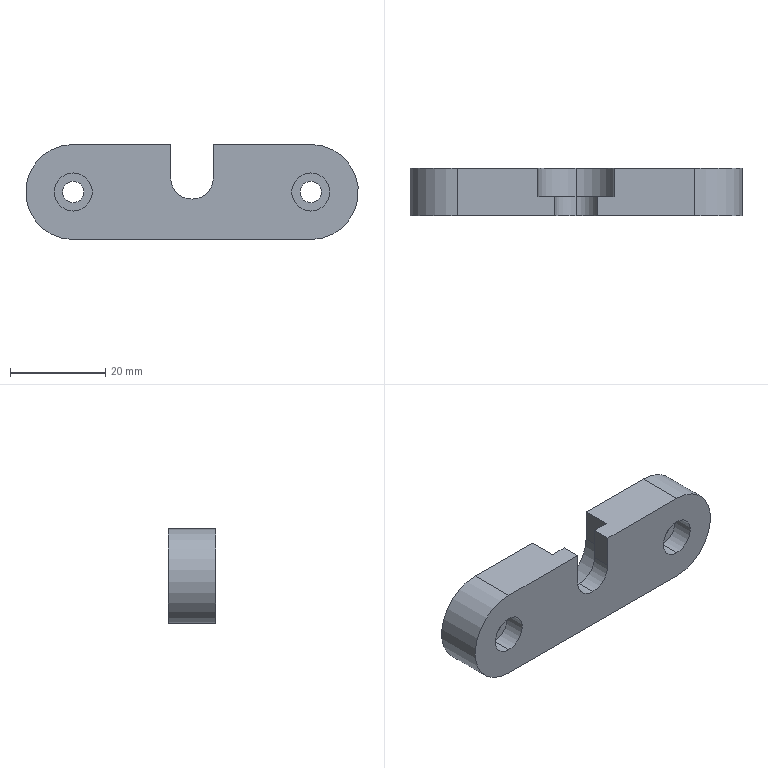Component | SolidWorks | 002MaterialPickingModuleA-1_004SidePlugModule-1_J-018-1 | 1 solid | 26 faces | box 70 x 10 x 20 mm | volume 10867 mm3 | cylinder 14 | plane 12 | commonest cylinder face diameters 8 x4 4.5 x4 9 x2 16 x2 20 x2 | material 45
build123d program:
from build123d import *

# Parameters (mm, degrees)
BOSS_EXTRUDE1_DEPTH                             = 5
M4_HEX_SOCKET_HEAD_CAP_SCREW_CBORE1_D           = 4.5
M4_HEX_SOCKET_HEAD_CAP_SCREW_CBORE1_CBORE_D     = 8
M4_HEX_SOCKET_HEAD_CAP_SCREW_CBORE1_CBORE_DEPTH = 4.4
CUT_EXTRUDE1_DEPTH                              = 6
CUT_EXTRUDE2_DEPTH                              = 37.892


with BuildPart() as part:
    # Sketch1 → Boss-Extrude1 (new, symmetric)
    with BuildSketch(Plane(origin=(0, 0, 0), x_dir=(1, 0, 0), z_dir=(0, 1, 0))):
        with BuildLine():
            Line((25, -10), (-25, -10))
            ThreePointArc((-25, -10), (-35, 0), (-25, 10))
            Line((-25, 10), (25, 10))
            ThreePointArc((25, 10), (35, 0), (25, -10))
        make_face()
    extrude(amount=BOSS_EXTRUDE1_DEPTH, both=True)

    # M4 Hex Socket Head Cap Screw CBORE1 (through all)
    with Locations(Plane(origin=(0, 5, 0), x_dir=(1, 0, 0), z_dir=(0, 1, 0))):
        with Locations((-25, 0), (25, 0)):
            CounterBoreHole(M4_HEX_SOCKET_HEAD_CAP_SCREW_CBORE1_D / 2, M4_HEX_SOCKET_HEAD_CAP_SCREW_CBORE1_CBORE_D / 2, M4_HEX_SOCKET_HEAD_CAP_SCREW_CBORE1_CBORE_DEPTH)

    # Sketch4 → Cut-Extrude1 (cut)
    with BuildSketch(Plane.XZ.offset(5)):
        with BuildLine():
            Line((8, 10), (8, 3))
            ThreePointArc((8, 3), (0, -5), (-8, 3))
            Line((-8, 3), (-8, 10))
            ThreePointArc((-8, 10), (0, 18), (8, 10))
        make_face()
    extrude(amount=-CUT_EXTRUDE1_DEPTH, mode=Mode.SUBTRACT)

    # Sketch5 → Cut-Extrude2 (cut, through all)
    with BuildSketch(Plane.XZ.offset(-1)):
        with BuildLine():
            Line((-4.5, 3), (-4.5, 10))
            ThreePointArc((-4.5, 10), (0, 14.5), (4.5, 10))
            Line((4.5, 10), (4.5, 3))
            ThreePointArc((4.5, 3), (0, -1.5), (-4.5, 3))
        make_face()
    extrude(amount=-CUT_EXTRUDE2_DEPTH, mode=Mode.SUBTRACT)


solid = part.part

# Placed as in the assembly
solid = solid.moved(Location((220.325, 273.019, 464.731), (0, 0, 180)))
STEP:
#1=COLOUR_RGB('',0.7922,0.8196,0.9333);
#2=FILL_AREA_STYLE_COLOUR('',#1);
#3=FILL_AREA_STYLE('',(#2));
#4=SURFACE_STYLE_FILL_AREA(#3);
#5=SURFACE_SIDE_STYLE('',(#4));
#6=SURFACE_STYLE_USAGE(.BOTH.,#5);
#7=PRESENTATION_STYLE_ASSIGNMENT((#6));
#8=CARTESIAN_POINT('',(8.674,10.552,18.237));
#9=VERTEX_POINT('',#8);
#10=CARTESIAN_POINT('',(8.497,10.552,18.415));
#11=VERTEX_POINT('',#10);
#12=CARTESIAN_POINT('',(8.674,10.552,18.415));
#13=DIRECTION('',(0.,1.,0.));
#14=DIRECTION('',(0.,0.,-1.));
#15=AXIS2_PLACEMENT_3D('',#12,#13,#14);
#16=CIRCLE('',#15,0.1772);
#17=EDGE_CURVE('',#9,#11,#16,.T.);
#18=ORIENTED_EDGE('',*,*,#17,.F.);
#19=CARTESIAN_POINT('',(8.674,10.709,18.237));
#20=VERTEX_POINT('',#19);
#21=CARTESIAN_POINT('',(8.674,10.552,18.237));
#22=DIRECTION('',(0.,1.,0.));
#23=VECTOR('',#22,39.37);
#24=LINE('',#21,#23);
#25=EDGE_CURVE('',#9,#20,#24,.T.);
#26=ORIENTED_EDGE('',*,*,#25,.T.);
#27=CARTESIAN_POINT('',(8.497,10.709,18.415));
#28=VERTEX_POINT('',#27);
#29=CARTESIAN_POINT('',(8.674,10.709,18.415));
#30=DIRECTION('',(0.,1.,0.));
#31=DIRECTION('',(0.,0.,-1.));
#32=AXIS2_PLACEMENT_3D('',#29,#30,#31);
#33=CIRCLE('',#32,0.1772);
#34=EDGE_CURVE('',#20,#28,#33,.T.);
#35=ORIENTED_EDGE('',*,*,#34,.T.);
#36=CARTESIAN_POINT('',(8.497,10.552,18.415));
#37=DIRECTION('',(0.,1.,0.));
#38=VECTOR('',#37,39.37);
#39=LINE('',#36,#38);
#40=EDGE_CURVE('',#11,#28,#39,.T.);
#41=ORIENTED_EDGE('',*,*,#40,.F.);
#42=EDGE_LOOP('',(#18,#26,#35,#41));
#43=FACE_OUTER_BOUND('',#42,.T.);
#44=CARTESIAN_POINT('',(8.674,10.552,18.415));
#45=DIRECTION('',(0.,1.,0.));
#46=DIRECTION('',(0.,0.,-1.));
#47=AXIS2_PLACEMENT_3D('',#44,#45,#46);
#48=CYLINDRICAL_SURFACE('',#47,0.1772);
#49=ADVANCED_FACE('',(#43),#48,.F.);
#50=CARTESIAN_POINT('',(8.674,10.709,18.1));
#51=VERTEX_POINT('',#50);
#52=CARTESIAN_POINT('',(8.359,10.709,18.415));
#53=VERTEX_POINT('',#52);
#54=CARTESIAN_POINT('',(8.674,10.709,18.415));
#55=DIRECTION('',(0.,1.,0.));
#56=DIRECTION('',(0.,0.,1.));
#57=AXIS2_PLACEMENT_3D('',#54,#55,#56);
#58=CIRCLE('',#57,0.315);
#59=EDGE_CURVE('',#51,#53,#58,.T.);
#60=ORIENTED_EDGE('',*,*,#59,.F.);
#61=CARTESIAN_POINT('',(8.674,10.946,18.1));
#62=VERTEX_POINT('',#61);
#63=CARTESIAN_POINT('',(8.674,9.449,18.1));
#64=DIRECTION('',(0.,1.,0.));
#65=VECTOR('',#64,39.37);
#66=LINE('',#63,#65);
#67=EDGE_CURVE('',#51,#62,#66,.T.);
#68=ORIENTED_EDGE('',*,*,#67,.T.);
#69=CARTESIAN_POINT('',(8.359,10.946,18.415));
#70=VERTEX_POINT('',#69);
#71=CARTESIAN_POINT('',(8.674,10.946,18.415));
#72=DIRECTION('',(0.,1.,0.));
#73=DIRECTION('',(0.,0.,-1.));
#74=AXIS2_PLACEMENT_3D('',#71,#72,#73);
#75=CIRCLE('',#74,0.315);
#76=EDGE_CURVE('',#62,#70,#75,.T.);
#77=ORIENTED_EDGE('',*,*,#76,.T.);
#78=CARTESIAN_POINT('',(8.359,9.449,18.415));
#79=DIRECTION('',(0.,1.,0.));
#80=VECTOR('',#79,39.37);
#81=LINE('',#78,#80);
#82=EDGE_CURVE('',#53,#70,#81,.T.);
#83=ORIENTED_EDGE('',*,*,#82,.F.);
#84=EDGE_LOOP('',(#60,#68,#77,#83));
#85=FACE_OUTER_BOUND('',#84,.T.);
#86=CARTESIAN_POINT('',(8.674,9.449,18.415));
#87=DIRECTION('',(0.,1.,0.));
#88=DIRECTION('',(0.,0.,-1.));
#89=AXIS2_PLACEMENT_3D('',#86,#87,#88);
#90=CYLINDRICAL_SURFACE('',#89,0.315);
#91=ADVANCED_FACE('',(#85),#90,.F.);
#92=CARTESIAN_POINT('',(9.658,10.725,18.139));
#93=VERTEX_POINT('',#92);
#94=CARTESIAN_POINT('',(9.658,10.725,18.454));
#95=VERTEX_POINT('',#94);
#96=CARTESIAN_POINT('',(9.658,10.725,18.296));
#97=DIRECTION('',(-0.,-1.,-0.));
#98=DIRECTION('',(0.,0.,1.));
#99=AXIS2_PLACEMENT_3D('',#96,#97,#98);
#100=CIRCLE('',#99,0.1575);
#101=EDGE_CURVE('',#93,#95,#100,.T.);
#102=ORIENTED_EDGE('',*,*,#101,.F.);
#103=CARTESIAN_POINT('',(9.658,10.552,18.139));
#104=VERTEX_POINT('',#103);
#105=CARTESIAN_POINT('',(9.658,10.552,18.139));
#106=DIRECTION('',(-0.,-1.,-0.));
#107=VECTOR('',#106,39.37);
#108=LINE('',#105,#107);
#109=EDGE_CURVE('',#93,#104,#108,.T.);
#110=ORIENTED_EDGE('',*,*,#109,.T.);
#111=CARTESIAN_POINT('',(9.658,10.552,18.454));
#112=VERTEX_POINT('',#111);
#113=CARTESIAN_POINT('',(9.658,10.552,18.296));
#114=DIRECTION('',(-0.,-1.,-0.));
#115=DIRECTION('',(0.,0.,1.));
#116=AXIS2_PLACEMENT_3D('',#113,#114,#115);
#117=CIRCLE('',#116,0.1575);
#118=EDGE_CURVE('',#104,#112,#117,.T.);
#119=ORIENTED_EDGE('',*,*,#118,.T.);
#120=CARTESIAN_POINT('',(9.658,10.552,18.454));
#121=DIRECTION('',(-0.,-1.,-0.));
#122=VECTOR('',#121,39.37);
#123=LINE('',#120,#122);
#124=EDGE_CURVE('',#95,#112,#123,.T.);
#125=ORIENTED_EDGE('',*,*,#124,.F.);
#126=EDGE_LOOP('',(#102,#110,#119,#125));
#127=FACE_OUTER_BOUND('',#126,.T.);
#128=CARTESIAN_POINT('',(9.658,10.552,18.296));
#129=DIRECTION('',(-0.,-1.,-0.));
#130=DIRECTION('',(0.,0.,1.));
#131=AXIS2_PLACEMENT_3D('',#128,#129,#130);
#132=CYLINDRICAL_SURFACE('',#131,0.1575);
#133=ADVANCED_FACE('',(#127),#132,.F.);
#134=CARTESIAN_POINT('',(9.658,10.946,18.208));
#135=VERTEX_POINT('',#134);
#136=CARTESIAN_POINT('',(9.658,10.946,18.385));
#137=VERTEX_POINT('',#136);
#138=CARTESIAN_POINT('',(9.658,10.946,18.296));
#139=DIRECTION('',(-0.,-1.,-0.));
#140=DIRECTION('',(0.,0.,1.));
#141=AXIS2_PLACEMENT_3D('',#138,#139,#140);
#142=CIRCLE('',#141,0.08858);
#143=EDGE_CURVE('',#135,#137,#142,.T.);
#144=ORIENTED_EDGE('',*,*,#143,.F.);
#145=CARTESIAN_POINT('',(9.658,10.725,18.208));
#146=VERTEX_POINT('',#145);
#147=CARTESIAN_POINT('',(9.658,10.552,18.208));
#148=DIRECTION('',(-0.,-1.,-0.));
#149=VECTOR('',#148,39.37);
#150=LINE('',#147,#149);
#151=EDGE_CURVE('',#135,#146,#150,.T.);
#152=ORIENTED_EDGE('',*,*,#151,.T.);
#153=CARTESIAN_POINT('',(9.658,10.725,18.385));
#154=VERTEX_POINT('',#153);
#155=CARTESIAN_POINT('',(9.658,10.725,18.296));
#156=DIRECTION('',(-0.,-1.,-0.));
#157=DIRECTION('',(0.,0.,1.));
#158=AXIS2_PLACEMENT_3D('',#155,#156,#157);
#159=CIRCLE('',#158,0.08858);
#160=EDGE_CURVE('',#146,#154,#159,.T.);
#161=ORIENTED_EDGE('',*,*,#160,.T.);
#162=CARTESIAN_POINT('',(9.658,10.552,18.385));
#163=DIRECTION('',(-0.,-1.,-0.));
#164=VECTOR('',#163,39.37);
#165=LINE('',#162,#164);
#166=EDGE_CURVE('',#137,#154,#165,.T.);
#167=ORIENTED_EDGE('',*,*,#166,.F.);
#168=EDGE_LOOP('',(#144,#152,#161,#167));
#169=FACE_OUTER_BOUND('',#168,.T.);
#170=CARTESIAN_POINT('',(9.658,10.552,18.296));
#171=DIRECTION('',(-0.,-1.,-0.));
#172=DIRECTION('',(0.,0.,1.));
#173=AXIS2_PLACEMENT_3D('',#170,#171,#172);
#174=CYLINDRICAL_SURFACE('',#173,0.08858);
#175=ADVANCED_FACE('',(#169),#174,.F.);
#176=CARTESIAN_POINT('',(7.69,10.725,18.139));
#177=VERTEX_POINT('',#176);
#178=CARTESIAN_POINT('',(7.69,10.725,18.454));
#179=VERTEX_POINT('',#178);
#180=CARTESIAN_POINT('',(7.69,10.725,18.296));
#181=DIRECTION('',(-0.,-1.,-0.));
#182=DIRECTION('',(0.,0.,1.));
#183=AXIS2_PLACEMENT_3D('',#180,#181,#182);
#184=CIRCLE('',#183,0.1575);
#185=EDGE_CURVE('',#177,#179,#184,.T.);
#186=ORIENTED_EDGE('',*,*,#185,.F.);
#187=CARTESIAN_POINT('',(7.69,10.552,18.139));
#188=VERTEX_POINT('',#187);
#189=CARTESIAN_POINT('',(7.69,10.552,18.139));
#190=DIRECTION('',(-0.,-1.,-0.));
#191=VECTOR('',#190,39.37);
#192=LINE('',#189,#191);
#193=EDGE_CURVE('',#177,#188,#192,.T.);
#194=ORIENTED_EDGE('',*,*,#193,.T.);
#195=CARTESIAN_POINT('',(7.69,10.552,18.454));
#196=VERTEX_POINT('',#195);
#197=CARTESIAN_POINT('',(7.69,10.552,18.296));
#198=DIRECTION('',(-0.,-1.,-0.));
#199=DIRECTION('',(0.,0.,1.));
#200=AXIS2_PLACEMENT_3D('',#197,#198,#199);
#201=CIRCLE('',#200,0.1575);
#202=EDGE_CURVE('',#188,#196,#201,.T.);
#203=ORIENTED_EDGE('',*,*,#202,.T.);
#204=CARTESIAN_POINT('',(7.69,10.552,18.454));
#205=DIRECTION('',(-0.,-1.,-0.));
#206=VECTOR('',#205,39.37);
#207=LINE('',#204,#206);
#208=EDGE_CURVE('',#179,#196,#207,.T.);
#209=ORIENTED_EDGE('',*,*,#208,.F.);
#210=EDGE_LOOP('',(#186,#194,#203,#209));
#211=FACE_OUTER_BOUND('',#210,.T.);
#212=CARTESIAN_POINT('',(7.69,10.552,18.296));
#213=DIRECTION('',(-0.,-1.,-0.));
#214=DIRECTION('',(0.,0.,1.));
#215=AXIS2_PLACEMENT_3D('',#212,#213,#214);
#216=CYLINDRICAL_SURFACE('',#215,0.1575);
#217=ADVANCED_FACE('',(#211),#216,.F.);
#218=CARTESIAN_POINT('',(7.69,10.946,18.208));
#219=VERTEX_POINT('',#218);
#220=CARTESIAN_POINT('',(7.69,10.946,18.385));
#221=VERTEX_POINT('',#220);
#222=CARTESIAN_POINT('',(7.69,10.946,18.296));
#223=DIRECTION('',(-0.,-1.,-0.));
#224=DIRECTION('',(0.,0.,1.));
#225=AXIS2_PLACEMENT_3D('',#222,#223,#224);
#226=CIRCLE('',#225,0.08858);
#227=EDGE_CURVE('',#219,#221,#226,.T.);
#228=ORIENTED_EDGE('',*,*,#227,.F.);
#229=CARTESIAN_POINT('',(7.69,10.725,18.208));
#230=VERTEX_POINT('',#229);
#231=CARTESIAN_POINT('',(7.69,10.552,18.208));
#232=DIRECTION('',(-0.,-1.,-0.));
#233=VECTOR('',#232,39.37);
#234=LINE('',#231,#233);
#235=EDGE_CURVE('',#219,#230,#234,.T.);
#236=ORIENTED_EDGE('',*,*,#235,.T.);
#237=CARTESIAN_POINT('',(7.69,10.725,18.385));
#238=VERTEX_POINT('',#237);
#239=CARTESIAN_POINT('',(7.69,10.725,18.296));
#240=DIRECTION('',(-0.,-1.,-0.));
#241=DIRECTION('',(0.,0.,1.));
#242=AXIS2_PLACEMENT_3D('',#239,#240,#241);
#243=CIRCLE('',#242,0.08858);
#244=EDGE_CURVE('',#230,#238,#243,.T.);
#245=ORIENTED_EDGE('',*,*,#244,.T.);
#246=CARTESIAN_POINT('',(7.69,10.552,18.385));
#247=DIRECTION('',(-0.,-1.,-0.));
#248=VECTOR('',#247,39.37);
#249=LINE('',#246,#248);
#250=EDGE_CURVE('',#221,#238,#249,.T.);
#251=ORIENTED_EDGE('',*,*,#250,.F.);
#252=EDGE_LOOP('',(#228,#236,#245,#251));
#253=FACE_OUTER_BOUND('',#252,.T.);
#254=CARTESIAN_POINT('',(7.69,10.552,18.296));
#255=DIRECTION('',(-0.,-1.,-0.));
#256=DIRECTION('',(0.,0.,1.));
#257=AXIS2_PLACEMENT_3D('',#254,#255,#256);
#258=CYLINDRICAL_SURFACE('',#257,0.08858);
#259=ADVANCED_FACE('',(#253),#258,.F.);
#260=CARTESIAN_POINT('',(8.989,10.709,18.69));
#261=VERTEX_POINT('',#260);
#262=CARTESIAN_POINT('',(8.851,10.709,18.69));
#263=VERTEX_POINT('',#262);
#264=CARTESIAN_POINT('',(7.69,10.709,18.69));
#265=DIRECTION('',(-1.,0.,-0.));
#266=VECTOR('',#265,39.37);
#267=LINE('',#264,#266);
#268=EDGE_CURVE('',#261,#263,#267,.T.);
#269=ORIENTED_EDGE('',*,*,#268,.T.);
#270=CARTESIAN_POINT('',(8.851,10.552,18.69));
#271=VERTEX_POINT('',#270);
#272=CARTESIAN_POINT('',(8.851,10.552,18.69));
#273=DIRECTION('',(0.,1.,0.));
#274=VECTOR('',#273,39.37);
#275=LINE('',#272,#274);
#276=EDGE_CURVE('',#271,#263,#275,.T.);
#277=ORIENTED_EDGE('',*,*,#276,.F.);
#278=CARTESIAN_POINT('',(9.658,10.552,18.69));
#279=VERTEX_POINT('',#278);
#280=CARTESIAN_POINT('',(7.69,10.552,18.69));
#281=DIRECTION('',(-1.,0.,-0.));
#282=VECTOR('',#281,39.37);
#283=LINE('',#280,#282);
#284=EDGE_CURVE('',#279,#271,#283,.T.);
#285=ORIENTED_EDGE('',*,*,#284,.F.);
#286=CARTESIAN_POINT('',(9.658,10.946,18.69));
#287=VERTEX_POINT('',#286);
#288=CARTESIAN_POINT('',(9.658,10.552,18.69));
#289=DIRECTION('',(0.,1.,0.));
#290=VECTOR('',#289,39.37);
#291=LINE('',#288,#290);
#292=EDGE_CURVE('',#279,#287,#291,.T.);
#293=ORIENTED_EDGE('',*,*,#292,.T.);
#294=CARTESIAN_POINT('',(8.989,10.946,18.69));
#295=VERTEX_POINT('',#294);
#296=CARTESIAN_POINT('',(7.69,10.946,18.69));
#297=DIRECTION('',(-1.,0.,-0.));
#298=VECTOR('',#297,39.37);
#299=LINE('',#296,#298);
#300=EDGE_CURVE('',#287,#295,#299,.T.);
#301=ORIENTED_EDGE('',*,*,#300,.T.);
#302=CARTESIAN_POINT('',(8.989,9.449,18.69));
#303=DIRECTION('',(0.,1.,0.));
#304=VECTOR('',#303,39.37);
#305=LINE('',#302,#304);
#306=EDGE_CURVE('',#261,#295,#305,.T.);
#307=ORIENTED_EDGE('',*,*,#306,.F.);
#308=EDGE_LOOP('',(#269,#277,#285,#293,#301,#307));
#309=FACE_OUTER_BOUND('',#308,.T.);
#310=CARTESIAN_POINT('',(7.69,10.552,18.69));
#311=DIRECTION('',(0.,0.,-1.));
#312=DIRECTION('',(1.,-0.,0.));
#313=AXIS2_PLACEMENT_3D('',#310,#311,#312);
#314=PLANE('',#313);
#315=ADVANCED_FACE('',(#309),#314,.F.);
#316=CARTESIAN_POINT('',(7.69,10.946,18.69));
#317=VERTEX_POINT('',#316);
#318=CARTESIAN_POINT('',(7.69,10.946,17.903));
#319=VERTEX_POINT('',#318);
#320=CARTESIAN_POINT('',(7.69,10.946,18.296));
#321=DIRECTION('',(-0.,-1.,-0.));
#322=DIRECTION('',(0.,0.,1.));
#323=AXIS2_PLACEMENT_3D('',#320,#321,#322);
#324=CIRCLE('',#323,0.3937);
#325=EDGE_CURVE('',#317,#319,#324,.T.);
#326=ORIENTED_EDGE('',*,*,#325,.T.);
#327=CARTESIAN_POINT('',(7.69,10.552,17.903));
#328=VERTEX_POINT('',#327);
#329=CARTESIAN_POINT('',(7.69,10.552,17.903));
#330=DIRECTION('',(0.,1.,0.));
#331=VECTOR('',#330,39.37);
#332=LINE('',#329,#331);
#333=EDGE_CURVE('',#328,#319,#332,.T.);
#334=ORIENTED_EDGE('',*,*,#333,.F.);
#335=CARTESIAN_POINT('',(7.69,10.552,18.69));
#336=VERTEX_POINT('',#335);
#337=CARTESIAN_POINT('',(7.69,10.552,18.296));
#338=DIRECTION('',(-0.,-1.,-0.));
#339=DIRECTION('',(0.,0.,1.));
#340=AXIS2_PLACEMENT_3D('',#337,#338,#339);
#341=CIRCLE('',#340,0.3937);
#342=EDGE_CURVE('',#336,#328,#341,.T.);
#343=ORIENTED_EDGE('',*,*,#342,.F.);
#344=CARTESIAN_POINT('',(7.69,10.552,18.69));
#345=DIRECTION('',(0.,1.,0.));
#346=VECTOR('',#345,39.37);
#347=LINE('',#344,#346);
#348=EDGE_CURVE('',#336,#317,#347,.T.);
#349=ORIENTED_EDGE('',*,*,#348,.T.);
#350=EDGE_LOOP('',(#326,#334,#343,#349));
#351=FACE_OUTER_BOUND('',#350,.T.);
#352=CARTESIAN_POINT('',(7.69,10.552,18.296));
#353=DIRECTION('',(0.,1.,0.));
#354=DIRECTION('',(0.,0.,-1.));
#355=AXIS2_PLACEMENT_3D('',#352,#353,#354);
#356=CYLINDRICAL_SURFACE('',#355,0.3937);
#357=ADVANCED_FACE('',(#351),#356,.T.);
#358=CARTESIAN_POINT('',(9.658,10.946,17.903));
#359=VERTEX_POINT('',#358);
#360=CARTESIAN_POINT('',(7.69,10.946,17.903));
#361=DIRECTION('',(1.,-0.,0.));
#362=VECTOR('',#361,39.37);
#363=LINE('',#360,#362);
#364=EDGE_CURVE('',#319,#359,#363,.T.);
#365=ORIENTED_EDGE('',*,*,#364,.T.);
#366=CARTESIAN_POINT('',(9.658,10.552,17.903));
#367=VERTEX_POINT('',#366);
#368=CARTESIAN_POINT('',(9.658,10.552,17.903));
#369=DIRECTION('',(0.,1.,0.));
#370=VECTOR('',#369,39.37);
#371=LINE('',#368,#370);
#372=EDGE_CURVE('',#367,#359,#371,.T.);
#373=ORIENTED_EDGE('',*,*,#372,.F.);
#374=CARTESIAN_POINT('',(7.69,10.552,17.903));
#375=DIRECTION('',(1.,-0.,0.));
#376=VECTOR('',#375,39.37);
#377=LINE('',#374,#376);
#378=EDGE_CURVE('',#328,#367,#377,.T.);
#379=ORIENTED_EDGE('',*,*,#378,.F.);
#380=ORIENTED_EDGE('',*,*,#333,.T.);
#381=EDGE_LOOP('',(#365,#373,#379,#380));
#382=FACE_OUTER_BOUND('',#381,.T.);
#383=CARTESIAN_POINT('',(7.69,10.552,17.903));
#384=DIRECTION('',(-0.,-0.,1.));
#385=DIRECTION('',(-1.,0.,-0.));
#386=AXIS2_PLACEMENT_3D('',#383,#384,#385);
#387=PLANE('',#386);
#388=ADVANCED_FACE('',(#382),#387,.F.);
#389=CARTESIAN_POINT('',(9.658,10.946,18.296));
#390=DIRECTION('',(-0.,-1.,-0.));
#391=DIRECTION('',(0.,0.,1.));
#392=AXIS2_PLACEMENT_3D('',#389,#390,#391);
#393=CIRCLE('',#392,0.3937);
#394=EDGE_CURVE('',#359,#287,#393,.T.);
#395=ORIENTED_EDGE('',*,*,#394,.T.);
#396=ORIENTED_EDGE('',*,*,#292,.F.);
#397=CARTESIAN_POINT('',(9.658,10.552,18.296));
#398=DIRECTION('',(-0.,-1.,-0.));
#399=DIRECTION('',(0.,0.,1.));
#400=AXIS2_PLACEMENT_3D('',#397,#398,#399);
#401=CIRCLE('',#400,0.3937);
#402=EDGE_CURVE('',#367,#279,#401,.T.);
#403=ORIENTED_EDGE('',*,*,#402,.F.);
#404=ORIENTED_EDGE('',*,*,#372,.T.);
#405=EDGE_LOOP('',(#395,#396,#403,#404));
#406=FACE_OUTER_BOUND('',#405,.T.);
#407=CARTESIAN_POINT('',(9.658,10.552,18.296));
#408=DIRECTION('',(0.,1.,0.));
#409=DIRECTION('',(0.,0.,-1.));
#410=AXIS2_PLACEMENT_3D('',#407,#408,#409);
#411=CYLINDRICAL_SURFACE('',#410,0.3937);
#412=ADVANCED_FACE('',(#406),#411,.T.);
#413=CARTESIAN_POINT('',(8.497,10.552,18.69));
#414=VERTEX_POINT('',#413);
#415=CARTESIAN_POINT('',(7.69,10.552,18.69));
#416=DIRECTION('',(-1.,0.,-0.));
#417=VECTOR('',#416,39.37);
#418=LINE('',#415,#417);
#419=EDGE_CURVE('',#414,#336,#418,.T.);
#420=ORIENTED_EDGE('',*,*,#419,.F.);
#421=CARTESIAN_POINT('',(8.497,10.709,18.69));
#422=VERTEX_POINT('',#421);
#423=CARTESIAN_POINT('',(8.497,10.552,18.69));
#424=DIRECTION('',(0.,1.,0.));
#425=VECTOR('',#424,39.37);
#426=LINE('',#423,#425);
#427=EDGE_CURVE('',#414,#422,#426,.T.);
#428=ORIENTED_EDGE('',*,*,#427,.T.);
#429=CARTESIAN_POINT('',(8.359,10.709,18.69));
#430=VERTEX_POINT('',#429);
#431=CARTESIAN_POINT('',(7.69,10.709,18.69));
#432=DIRECTION('',(-1.,0.,-0.));
#433=VECTOR('',#432,39.37);
#434=LINE('',#431,#433);
#435=EDGE_CURVE('',#422,#430,#434,.T.);
#436=ORIENTED_EDGE('',*,*,#435,.T.);
#437=CARTESIAN_POINT('',(8.359,10.946,18.69));
#438=VERTEX_POINT('',#437);
#439=CARTESIAN_POINT('',(8.359,9.449,18.69));
#440=DIRECTION('',(0.,1.,0.));
#441=VECTOR('',#440,39.37);
#442=LINE('',#439,#441);
#443=EDGE_CURVE('',#430,#438,#442,.T.);
#444=ORIENTED_EDGE('',*,*,#443,.T.);
#445=CARTESIAN_POINT('',(7.69,10.946,18.69));
#446=DIRECTION('',(-1.,0.,-0.));
#447=VECTOR('',#446,39.37);
#448=LINE('',#445,#447);
#449=EDGE_CURVE('',#438,#317,#448,.T.);
#450=ORIENTED_EDGE('',*,*,#449,.T.);
#451=ORIENTED_EDGE('',*,*,#348,.F.);
#452=EDGE_LOOP('',(#420,#428,#436,#444,#450,#451));
#453=FACE_OUTER_BOUND('',#452,.T.);
#454=CARTESIAN_POINT('',(7.69,10.552,18.69));
#455=DIRECTION('',(0.,0.,-1.));
#456=DIRECTION('',(1.,-0.,0.));
#457=AXIS2_PLACEMENT_3D('',#454,#455,#456);
#458=PLANE('',#457);
#459=ADVANCED_FACE('',(#453),#458,.F.);
#460=CARTESIAN_POINT('',(8.851,10.552,18.415));
#461=VERTEX_POINT('',#460);
#462=CARTESIAN_POINT('',(8.851,10.552,18.415));
#463=DIRECTION('',(0.,0.,-1.));
#464=VECTOR('',#463,39.37);
#465=LINE('',#462,#464);
#466=EDGE_CURVE('',#271,#461,#465,.T.);
#467=ORIENTED_EDGE('',*,*,#466,.T.);
#468=CARTESIAN_POINT('',(8.674,10.552,18.415));
#469=DIRECTION('',(0.,1.,0.));
#470=DIRECTION('',(0.,0.,-1.));
#471=AXIS2_PLACEMENT_3D('',#468,#469,#470);
#472=CIRCLE('',#471,0.1772);
#473=EDGE_CURVE('',#461,#9,#472,.T.);
#474=ORIENTED_EDGE('',*,*,#473,.T.);
#475=ORIENTED_EDGE('',*,*,#17,.T.);
#476=CARTESIAN_POINT('',(8.497,10.552,18.415));
#477=DIRECTION('',(-0.,-0.,1.));
#478=VECTOR('',#477,39.37);
#479=LINE('',#476,#478);
#480=EDGE_CURVE('',#11,#414,#479,.T.);
#481=ORIENTED_EDGE('',*,*,#480,.T.);
#482=ORIENTED_EDGE('',*,*,#419,.T.);
#483=ORIENTED_EDGE('',*,*,#342,.T.);
#484=ORIENTED_EDGE('',*,*,#378,.T.);
#485=ORIENTED_EDGE('',*,*,#402,.T.);
#486=ORIENTED_EDGE('',*,*,#284,.T.);
#487=EDGE_LOOP('',(#467,#474,#475,#481,#482,#483,#484,#485,#486));
#488=FACE_OUTER_BOUND('',#487,.T.);
#489=CARTESIAN_POINT('',(9.658,10.552,18.296));
#490=DIRECTION('',(-0.,-1.,-0.));
#491=DIRECTION('',(0.,0.,1.));
#492=AXIS2_PLACEMENT_3D('',#489,#490,#491);
#493=CIRCLE('',#492,0.1575);
#494=EDGE_CURVE('',#112,#104,#493,.T.);
#495=ORIENTED_EDGE('',*,*,#494,.F.);
#496=ORIENTED_EDGE('',*,*,#118,.F.);
#497=EDGE_LOOP('',(#495,#496));
#498=FACE_BOUND('',#497,.T.);
#499=CARTESIAN_POINT('',(7.69,10.552,18.296));
#500=DIRECTION('',(-0.,-1.,-0.));
#501=DIRECTION('',(0.,0.,1.));
#502=AXIS2_PLACEMENT_3D('',#499,#500,#501);
#503=CIRCLE('',#502,0.1575);
#504=EDGE_CURVE('',#196,#188,#503,.T.);
#505=ORIENTED_EDGE('',*,*,#504,.F.);
#506=ORIENTED_EDGE('',*,*,#202,.F.);
#507=EDGE_LOOP('',(#505,#506));
#508=FACE_BOUND('',#507,.T.);
#509=CARTESIAN_POINT('',(7.69,10.552,18.296));
#510=DIRECTION('',(-0.,-1.,-0.));
#511=DIRECTION('',(-0.,-0.,1.));
#512=AXIS2_PLACEMENT_3D('',#509,#510,#511);
#513=PLANE('',#512);
#514=ADVANCED_FACE('',(#488,#498,#508),#513,.T.);
#515=CARTESIAN_POINT('',(9.658,10.946,18.296));
#516=DIRECTION('',(-0.,-1.,-0.));
#517=DIRECTION('',(0.,0.,1.));
#518=AXIS2_PLACEMENT_3D('',#515,#516,#517);
#519=CIRCLE('',#518,0.08858);
#520=EDGE_CURVE('',#137,#135,#519,.T.);
#521=ORIENTED_EDGE('',*,*,#520,.T.);
#522=ORIENTED_EDGE('',*,*,#143,.T.);
#523=EDGE_LOOP('',(#521,#522));
#524=FACE_BOUND('',#523,.T.);
#525=CARTESIAN_POINT('',(7.69,10.946,18.296));
#526=DIRECTION('',(-0.,-1.,-0.));
#527=DIRECTION('',(0.,0.,1.));
#528=AXIS2_PLACEMENT_3D('',#525,#526,#527);
#529=CIRCLE('',#528,0.08858);
#530=EDGE_CURVE('',#221,#219,#529,.T.);
#531=ORIENTED_EDGE('',*,*,#530,.T.);
#532=ORIENTED_EDGE('',*,*,#227,.T.);
#533=EDGE_LOOP('',(#531,#532));
#534=FACE_BOUND('',#533,.T.);
#535=CARTESIAN_POINT('',(8.989,10.946,18.415));
#536=VERTEX_POINT('',#535);
#537=CARTESIAN_POINT('',(8.674,10.946,18.415));
#538=DIRECTION('',(0.,1.,0.));
#539=DIRECTION('',(0.,0.,-1.));
#540=AXIS2_PLACEMENT_3D('',#537,#538,#539);
#541=CIRCLE('',#540,0.315);
#542=EDGE_CURVE('',#536,#62,#541,.T.);
#543=ORIENTED_EDGE('',*,*,#542,.F.);
#544=CARTESIAN_POINT('',(8.989,10.946,18.69));
#545=DIRECTION('',(-0.,0.,-1.));
#546=VECTOR('',#545,39.37);
#547=LINE('',#544,#546);
#548=EDGE_CURVE('',#295,#536,#547,.T.);
#549=ORIENTED_EDGE('',*,*,#548,.F.);
#550=ORIENTED_EDGE('',*,*,#300,.F.);
#551=ORIENTED_EDGE('',*,*,#394,.F.);
#552=ORIENTED_EDGE('',*,*,#364,.F.);
#553=ORIENTED_EDGE('',*,*,#325,.F.);
#554=ORIENTED_EDGE('',*,*,#449,.F.);
#555=CARTESIAN_POINT('',(8.359,10.946,18.69));
#556=DIRECTION('',(0.,-0.,1.));
#557=VECTOR('',#556,39.37);
#558=LINE('',#555,#557);
#559=EDGE_CURVE('',#70,#438,#558,.T.);
#560=ORIENTED_EDGE('',*,*,#559,.F.);
#561=ORIENTED_EDGE('',*,*,#76,.F.);
#562=EDGE_LOOP('',(#543,#549,#550,#551,#552,#553,#554,#560,#561));
#563=FACE_OUTER_BOUND('',#562,.T.);
#564=CARTESIAN_POINT('',(7.69,10.946,18.296));
#565=DIRECTION('',(-0.,-1.,-0.));
#566=DIRECTION('',(-0.,-0.,1.));
#567=AXIS2_PLACEMENT_3D('',#564,#565,#566);
#568=PLANE('',#567);
#569=ADVANCED_FACE('',(#524,#534,#563),#568,.F.);
#570=ORIENTED_EDGE('',*,*,#235,.F.);
#571=ORIENTED_EDGE('',*,*,#530,.F.);
#572=ORIENTED_EDGE('',*,*,#250,.T.);
#573=CARTESIAN_POINT('',(7.69,10.725,18.296));
#574=DIRECTION('',(-0.,-1.,-0.));
#575=DIRECTION('',(0.,0.,1.));
#576=AXIS2_PLACEMENT_3D('',#573,#574,#575);
#577=CIRCLE('',#576,0.08858);
#578=EDGE_CURVE('',#238,#230,#577,.T.);
#579=ORIENTED_EDGE('',*,*,#578,.T.);
#580=EDGE_LOOP('',(#570,#571,#572,#579));
#581=FACE_OUTER_BOUND('',#580,.T.);
#582=CARTESIAN_POINT('',(7.69,10.552,18.296));
#583=DIRECTION('',(-0.,-1.,-0.));
#584=DIRECTION('',(0.,0.,1.));
#585=AXIS2_PLACEMENT_3D('',#582,#583,#584);
#586=CYLINDRICAL_SURFACE('',#585,0.08858);
#587=ADVANCED_FACE('',(#581),#586,.F.);
#588=ORIENTED_EDGE('',*,*,#578,.F.);
#589=ORIENTED_EDGE('',*,*,#244,.F.);
#590=EDGE_LOOP('',(#588,#589));
#591=FACE_BOUND('',#590,.T.);
#592=CARTESIAN_POINT('',(7.69,10.725,18.296));
#593=DIRECTION('',(-0.,-1.,-0.));
#594=DIRECTION('',(0.,0.,1.));
#595=AXIS2_PLACEMENT_3D('',#592,#593,#594);
#596=CIRCLE('',#595,0.1575);
#597=EDGE_CURVE('',#179,#177,#596,.T.);
#598=ORIENTED_EDGE('',*,*,#597,.T.);
#599=ORIENTED_EDGE('',*,*,#185,.T.);
#600=EDGE_LOOP('',(#598,#599));
#601=FACE_OUTER_BOUND('',#600,.T.);
#602=CARTESIAN_POINT('',(7.601,10.725,18.296));
#603=DIRECTION('',(0.,1.,0.));
#604=DIRECTION('',(0.,0.,-1.));
#605=AXIS2_PLACEMENT_3D('',#602,#603,#604);
#606=PLANE('',#605);
#607=ADVANCED_FACE('',(#591,#601),#606,.F.);
#608=ORIENTED_EDGE('',*,*,#193,.F.);
#609=ORIENTED_EDGE('',*,*,#597,.F.);
#610=ORIENTED_EDGE('',*,*,#208,.T.);
#611=ORIENTED_EDGE('',*,*,#504,.T.);
#612=EDGE_LOOP('',(#608,#609,#610,#611));
#613=FACE_OUTER_BOUND('',#612,.T.);
#614=CARTESIAN_POINT('',(7.69,10.552,18.296));
#615=DIRECTION('',(-0.,-1.,-0.));
#616=DIRECTION('',(0.,0.,1.));
#617=AXIS2_PLACEMENT_3D('',#614,#615,#616);
#618=CYLINDRICAL_SURFACE('',#617,0.1575);
#619=ADVANCED_FACE('',(#613),#618,.F.);
#620=ORIENTED_EDGE('',*,*,#151,.F.);
#621=ORIENTED_EDGE('',*,*,#520,.F.);
#622=ORIENTED_EDGE('',*,*,#166,.T.);
#623=CARTESIAN_POINT('',(9.658,10.725,18.296));
#624=DIRECTION('',(-0.,-1.,-0.));
#625=DIRECTION('',(0.,0.,1.));
#626=AXIS2_PLACEMENT_3D('',#623,#624,#625);
#627=CIRCLE('',#626,0.08858);
#628=EDGE_CURVE('',#154,#146,#627,.T.);
#629=ORIENTED_EDGE('',*,*,#628,.T.);
#630=EDGE_LOOP('',(#620,#621,#622,#629));
#631=FACE_OUTER_BOUND('',#630,.T.);
#632=CARTESIAN_POINT('',(9.658,10.552,18.296));
#633=DIRECTION('',(-0.,-1.,-0.));
#634=DIRECTION('',(0.,0.,1.));
#635=AXIS2_PLACEMENT_3D('',#632,#633,#634);
#636=CYLINDRICAL_SURFACE('',#635,0.08858);
#637=ADVANCED_FACE('',(#631),#636,.F.);
#638=ORIENTED_EDGE('',*,*,#628,.F.);
#639=ORIENTED_EDGE('',*,*,#160,.F.);
#640=EDGE_LOOP('',(#638,#639));
#641=FACE_BOUND('',#640,.T.);
#642=CARTESIAN_POINT('',(9.658,10.725,18.296));
#643=DIRECTION('',(-0.,-1.,-0.));
#644=DIRECTION('',(0.,0.,1.));
#645=AXIS2_PLACEMENT_3D('',#642,#643,#644);
#646=CIRCLE('',#645,0.1575);
#647=EDGE_CURVE('',#95,#93,#646,.T.);
#648=ORIENTED_EDGE('',*,*,#647,.T.);
#649=ORIENTED_EDGE('',*,*,#101,.T.);
#650=EDGE_LOOP('',(#648,#649));
#651=FACE_OUTER_BOUND('',#650,.T.);
#652=CARTESIAN_POINT('',(9.57,10.725,18.296));
#653=DIRECTION('',(0.,1.,0.));
#654=DIRECTION('',(0.,0.,-1.));
#655=AXIS2_PLACEMENT_3D('',#652,#653,#654);
#656=PLANE('',#655);
#657=ADVANCED_FACE('',(#641,#651),#656,.F.);
#658=ORIENTED_EDGE('',*,*,#109,.F.);
#659=ORIENTED_EDGE('',*,*,#647,.F.);
#660=ORIENTED_EDGE('',*,*,#124,.T.);
#661=ORIENTED_EDGE('',*,*,#494,.T.);
#662=EDGE_LOOP('',(#658,#659,#660,#661));
#663=FACE_OUTER_BOUND('',#662,.T.);
#664=CARTESIAN_POINT('',(9.658,10.552,18.296));
#665=DIRECTION('',(-0.,-1.,-0.));
#666=DIRECTION('',(0.,0.,1.));
#667=AXIS2_PLACEMENT_3D('',#664,#665,#666);
#668=CYLINDRICAL_SURFACE('',#667,0.1575);
#669=ADVANCED_FACE('',(#663),#668,.F.);
#670=CARTESIAN_POINT('',(8.851,10.709,18.415));
#671=VERTEX_POINT('',#670);
#672=CARTESIAN_POINT('',(8.674,10.709,18.415));
#673=DIRECTION('',(0.,1.,0.));
#674=DIRECTION('',(0.,0.,-1.));
#675=AXIS2_PLACEMENT_3D('',#672,#673,#674);
#676=CIRCLE('',#675,0.1772);
#677=EDGE_CURVE('',#671,#20,#676,.T.);
#678=ORIENTED_EDGE('',*,*,#677,.F.);
#679=CARTESIAN_POINT('',(8.851,10.709,18.415));
#680=DIRECTION('',(0.,0.,-1.));
#681=VECTOR('',#680,39.37);
#682=LINE('',#679,#681);
#683=EDGE_CURVE('',#263,#671,#682,.T.);
#684=ORIENTED_EDGE('',*,*,#683,.F.);
#685=ORIENTED_EDGE('',*,*,#268,.F.);
#686=CARTESIAN_POINT('',(8.989,10.709,18.415));
#687=VERTEX_POINT('',#686);
#688=CARTESIAN_POINT('',(8.989,10.709,18.69));
#689=DIRECTION('',(-0.,0.,-1.));
#690=VECTOR('',#689,39.37);
#691=LINE('',#688,#690);
#692=EDGE_CURVE('',#261,#687,#691,.T.);
#693=ORIENTED_EDGE('',*,*,#692,.T.);
#694=CARTESIAN_POINT('',(8.674,10.709,18.415));
#695=DIRECTION('',(0.,1.,0.));
#696=DIRECTION('',(0.,0.,1.));
#697=AXIS2_PLACEMENT_3D('',#694,#695,#696);
#698=CIRCLE('',#697,0.315);
#699=EDGE_CURVE('',#687,#51,#698,.T.);
#700=ORIENTED_EDGE('',*,*,#699,.T.);
#701=ORIENTED_EDGE('',*,*,#59,.T.);
#702=CARTESIAN_POINT('',(8.359,10.709,18.69));
#703=DIRECTION('',(0.,-0.,1.));
#704=VECTOR('',#703,39.37);
#705=LINE('',#702,#704);
#706=EDGE_CURVE('',#53,#430,#705,.T.);
#707=ORIENTED_EDGE('',*,*,#706,.T.);
#708=ORIENTED_EDGE('',*,*,#435,.F.);
#709=CARTESIAN_POINT('',(8.497,10.709,18.415));
#710=DIRECTION('',(-0.,-0.,1.));
#711=VECTOR('',#710,39.37);
#712=LINE('',#709,#711);
#713=EDGE_CURVE('',#28,#422,#712,.T.);
#714=ORIENTED_EDGE('',*,*,#713,.F.);
#715=ORIENTED_EDGE('',*,*,#34,.F.);
#716=EDGE_LOOP('',(#678,#684,#685,#693,#700,#701,#707,#708,#714,#715));
#717=FACE_OUTER_BOUND('',#716,.T.);
#718=CARTESIAN_POINT('',(7.69,10.709,18.296));
#719=DIRECTION('',(-0.,-1.,-0.));
#720=DIRECTION('',(-0.,-0.,1.));
#721=AXIS2_PLACEMENT_3D('',#718,#719,#720);
#722=PLANE('',#721);
#723=ADVANCED_FACE('',(#717),#722,.F.);
#724=ORIENTED_EDGE('',*,*,#306,.T.);
#725=ORIENTED_EDGE('',*,*,#548,.T.);
#726=CARTESIAN_POINT('',(8.989,9.449,18.415));
#727=DIRECTION('',(0.,1.,0.));
#728=VECTOR('',#727,39.37);
#729=LINE('',#726,#728);
#730=EDGE_CURVE('',#687,#536,#729,.T.);
#731=ORIENTED_EDGE('',*,*,#730,.F.);
#732=ORIENTED_EDGE('',*,*,#692,.F.);
#733=EDGE_LOOP('',(#724,#725,#731,#732));
#734=FACE_OUTER_BOUND('',#733,.T.);
#735=CARTESIAN_POINT('',(8.989,9.449,18.69));
#736=DIRECTION('',(1.,-0.,-0.));
#737=DIRECTION('',(0.,-0.,1.));
#738=AXIS2_PLACEMENT_3D('',#735,#736,#737);
#739=PLANE('',#738);
#740=ADVANCED_FACE('',(#734),#739,.F.);
#741=ORIENTED_EDGE('',*,*,#67,.F.);
#742=ORIENTED_EDGE('',*,*,#699,.F.);
#743=ORIENTED_EDGE('',*,*,#730,.T.);
#744=ORIENTED_EDGE('',*,*,#542,.T.);
#745=EDGE_LOOP('',(#741,#742,#743,#744));
#746=FACE_OUTER_BOUND('',#745,.T.);
#747=CARTESIAN_POINT('',(8.674,9.449,18.415));
#748=DIRECTION('',(0.,1.,0.));
#749=DIRECTION('',(0.,0.,-1.));
#750=AXIS2_PLACEMENT_3D('',#747,#748,#749);
#751=CYLINDRICAL_SURFACE('',#750,0.315);
#752=ADVANCED_FACE('',(#746),#751,.F.);
#753=ORIENTED_EDGE('',*,*,#82,.T.);
#754=ORIENTED_EDGE('',*,*,#559,.T.);
#755=ORIENTED_EDGE('',*,*,#443,.F.);
#756=ORIENTED_EDGE('',*,*,#706,.F.);
#757=EDGE_LOOP('',(#753,#754,#755,#756));
#758=FACE_OUTER_BOUND('',#757,.T.);
#759=CARTESIAN_POINT('',(8.359,9.449,18.69));
#760=DIRECTION('',(-1.,0.,0.));
#761=DIRECTION('',(-0.,0.,-1.));
#762=AXIS2_PLACEMENT_3D('',#759,#760,#761);
#763=PLANE('',#762);
#764=ADVANCED_FACE('',(#758),#763,.F.);
#765=ORIENTED_EDGE('',*,*,#25,.F.);
#766=ORIENTED_EDGE('',*,*,#473,.F.);
#767=CARTESIAN_POINT('',(8.851,10.552,18.415));
#768=DIRECTION('',(0.,1.,0.));
#769=VECTOR('',#768,39.37);
#770=LINE('',#767,#769);
#771=EDGE_CURVE('',#461,#671,#770,.T.);
#772=ORIENTED_EDGE('',*,*,#771,.T.);
#773=ORIENTED_EDGE('',*,*,#677,.T.);
#774=EDGE_LOOP('',(#765,#766,#772,#773));
#775=FACE_OUTER_BOUND('',#774,.T.);
#776=CARTESIAN_POINT('',(8.674,10.552,18.415));
#777=DIRECTION('',(0.,1.,0.));
#778=DIRECTION('',(0.,0.,-1.));
#779=AXIS2_PLACEMENT_3D('',#776,#777,#778);
#780=CYLINDRICAL_SURFACE('',#779,0.1772);
#781=ADVANCED_FACE('',(#775),#780,.F.);
#782=ORIENTED_EDGE('',*,*,#683,.T.);
#783=ORIENTED_EDGE('',*,*,#771,.F.);
#784=ORIENTED_EDGE('',*,*,#466,.F.);
#785=ORIENTED_EDGE('',*,*,#276,.T.);
#786=EDGE_LOOP('',(#782,#783,#784,#785));
#787=FACE_OUTER_BOUND('',#786,.T.);
#788=CARTESIAN_POINT('',(8.851,10.552,18.415));
#789=DIRECTION('',(1.,-0.,0.));
#790=DIRECTION('',(-0.,-0.,1.));
#791=AXIS2_PLACEMENT_3D('',#788,#789,#790);
#792=PLANE('',#791);
#793=ADVANCED_FACE('',(#787),#792,.F.);
#794=ORIENTED_EDGE('',*,*,#713,.T.);
#795=ORIENTED_EDGE('',*,*,#427,.F.);
#796=ORIENTED_EDGE('',*,*,#480,.F.);
#797=ORIENTED_EDGE('',*,*,#40,.T.);
#798=EDGE_LOOP('',(#794,#795,#796,#797));
#799=FACE_OUTER_BOUND('',#798,.T.);
#800=CARTESIAN_POINT('',(8.497,10.552,18.415));
#801=DIRECTION('',(-1.,0.,-0.));
#802=DIRECTION('',(0.,0.,-1.));
#803=AXIS2_PLACEMENT_3D('',#800,#801,#802);
#804=PLANE('',#803);
#805=ADVANCED_FACE('',(#799),#804,.F.);
#806=CLOSED_SHELL('',(#49,#91,#133,#175,#217,#259,#315,#357,#388,#412,#459,#514,#569,#587,#607,#619,#637,#657,#669,#723,#740,#752,#764,#781,#793,#805));
#807=MANIFOLD_SOLID_BREP('',#806);
#808=STYLED_ITEM('',(#7),#807);
#809=PRESENTATION_LAYER_ASSIGNMENT('','',(#808));
#810=CARTESIAN_POINT('',(0.,0.,0.));
#811=DIRECTION('',(0.,0.,1.));
#812=DIRECTION('',(1.,0.,0.));
#813=AXIS2_PLACEMENT_3D('',#810,#811,#812);
#814=(LENGTH_UNIT()NAMED_UNIT(*)SI_UNIT($,.METRE.));
#815=LENGTH_MEASURE_WITH_UNIT(LENGTH_MEASURE(0.0254),#814);
#816=DIMENSIONAL_EXPONENTS(1.,0.,0.,0.,0.,0.,0.);
#817=(CONVERSION_BASED_UNIT('',#815)LENGTH_UNIT()NAMED_UNIT(#816));
#818=UNCERTAINTY_MEASURE_WITH_UNIT(LENGTH_MEASURE(0.00001),#817,'','');
#819=(NAMED_UNIT(*)PLANE_ANGLE_UNIT()SI_UNIT($,.RADIAN.));
#820=(NAMED_UNIT(*)SI_UNIT($,.STERADIAN.)SOLID_ANGLE_UNIT());
#821=(GEOMETRIC_REPRESENTATION_CONTEXT(3)GLOBAL_UNCERTAINTY_ASSIGNED_CONTEXT((#818))GLOBAL_UNIT_ASSIGNED_CONTEXT((#817,#819,#820))REPRESENTATION_CONTEXT('',''));
#822=ADVANCED_BREP_SHAPE_REPRESENTATION('',(#807,#813),#821);
#823=(LENGTH_UNIT()NAMED_UNIT(*)SI_UNIT($,.METRE.));
#824=LENGTH_MEASURE_WITH_UNIT(LENGTH_MEASURE(0.0254),#823);
#825=DIMENSIONAL_EXPONENTS(1.,0.,0.,0.,0.,0.,0.);
#826=(CONVERSION_BASED_UNIT('',#824)LENGTH_UNIT()NAMED_UNIT(#825));
#827=UNCERTAINTY_MEASURE_WITH_UNIT(LENGTH_MEASURE(0.00001),#826,'','');
#828=(NAMED_UNIT(*)PLANE_ANGLE_UNIT()SI_UNIT($,.RADIAN.));
#829=(NAMED_UNIT(*)SI_UNIT($,.STERADIAN.)SOLID_ANGLE_UNIT());
#830=(GEOMETRIC_REPRESENTATION_CONTEXT(3)GLOBAL_UNCERTAINTY_ASSIGNED_CONTEXT((#827))GLOBAL_UNIT_ASSIGNED_CONTEXT((#826,#828,#829))REPRESENTATION_CONTEXT('',''));
#831=MECHANICAL_DESIGN_GEOMETRIC_PRESENTATION_REPRESENTATION('',(#808),#830);